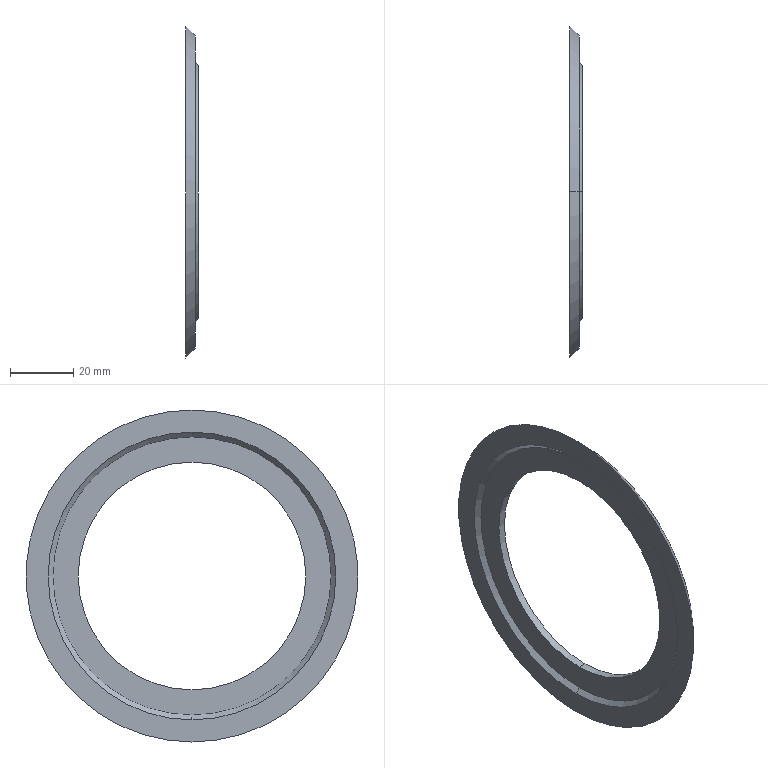Component | SolidWorks | 24Gasket-1 | 1 solid | 12 faces | box 4 x 105 x 105 mm | volume 10058 mm3 | cone 6 | plane 4 | cylinder 2 | commonest cylinder face diameters 72 x2
build123d program:
from build123d import *


with BuildPart() as part:
    # Sketch28 → Revolve1 (revolve)
    with BuildSketch(Plane(origin=(0, 0, 0), x_dir=(0, 0, -1), z_dir=(1, 0, 0)), mode=Mode.PRIVATE) as revolve1_sk:
        Polygon((0, 36), (0, 40), (-1, 41), (-1, 49.5), (-4, 52.5), (-4, 45.5), (-2.5, 44), (-2.5, 36), align=None)
    revolve(revolve1_sk.sketch.rotate(Axis((0, 0, 0), (0, 0, 1)), 90), axis=Axis((0, 0, 0), (0, 0, 1)))


solid = part.part

# Placed as in the assembly
solid = solid.moved(Location((-61.043, 1.776, 250), (0, -90, 0)))
STEP:
#1=CARTESIAN_POINT('',(-2.502,0.06992,11.575));
#2=VERTEX_POINT('',#1);
#3=CARTESIAN_POINT('',(-2.502,0.06992,8.11));
#4=VERTEX_POINT('',#3);
#5=CARTESIAN_POINT('',(-2.502,0.06992,9.843));
#6=DIRECTION('',(1.,0.,0.));
#7=DIRECTION('',(0.,0.,-1.));
#8=AXIS2_PLACEMENT_3D('',#5,#6,#7);
#9=CIRCLE('',#8,1.732);
#10=EDGE_CURVE('',#2,#4,#9,.T.);
#11=ORIENTED_EDGE('',*,*,#10,.T.);
#12=CARTESIAN_POINT('',(-2.561,0.06992,8.051));
#13=VERTEX_POINT('',#12);
#14=CARTESIAN_POINT('',(-2.561,0.06992,8.051));
#15=DIRECTION('',(-0.7071,0.,-0.7071));
#16=VECTOR('',#15,39.37);
#17=LINE('',#14,#16);
#18=EDGE_CURVE('',#4,#13,#17,.T.);
#19=ORIENTED_EDGE('',*,*,#18,.T.);
#20=CARTESIAN_POINT('',(-2.561,0.06992,11.634));
#21=VERTEX_POINT('',#20);
#22=CARTESIAN_POINT('',(-2.561,0.06992,9.843));
#23=DIRECTION('',(1.,0.,0.));
#24=DIRECTION('',(0.,0.,-1.));
#25=AXIS2_PLACEMENT_3D('',#22,#23,#24);
#26=CIRCLE('',#25,1.791);
#27=EDGE_CURVE('',#21,#13,#26,.T.);
#28=ORIENTED_EDGE('',*,*,#27,.F.);
#29=CARTESIAN_POINT('',(-2.561,0.06992,11.634));
#30=DIRECTION('',(-0.7071,0.,0.7071));
#31=VECTOR('',#30,39.37);
#32=LINE('',#29,#31);
#33=EDGE_CURVE('',#2,#21,#32,.T.);
#34=ORIENTED_EDGE('',*,*,#33,.F.);
#35=EDGE_LOOP('',(#11,#19,#28,#34));
#36=FACE_OUTER_BOUND('',#35,.T.);
#37=CARTESIAN_POINT('',(-2.561,0.06992,9.843));
#38=DIRECTION('',(-1.,-0.,-0.));
#39=DIRECTION('',(0.,0.,1.));
#40=AXIS2_PLACEMENT_3D('',#37,#38,#39);
#41=CONICAL_SURFACE('',#40,1.791,0.7854);
#42=ADVANCED_FACE('',(#36),#41,.F.);
#43=CARTESIAN_POINT('',(-2.443,0.06992,7.894));
#44=VERTEX_POINT('',#43);
#45=CARTESIAN_POINT('',(-2.443,0.06992,11.791));
#46=VERTEX_POINT('',#45);
#47=CARTESIAN_POINT('',(-2.443,0.06992,9.843));
#48=DIRECTION('',(1.,0.,0.));
#49=DIRECTION('',(0.,0.,-1.));
#50=AXIS2_PLACEMENT_3D('',#47,#48,#49);
#51=CIRCLE('',#50,1.949);
#52=EDGE_CURVE('',#44,#46,#51,.T.);
#53=ORIENTED_EDGE('',*,*,#52,.F.);
#54=CARTESIAN_POINT('',(-2.561,0.06992,7.776));
#55=VERTEX_POINT('',#54);
#56=CARTESIAN_POINT('',(-2.443,0.06992,7.894));
#57=DIRECTION('',(-0.7071,0.,-0.7071));
#58=VECTOR('',#57,39.37);
#59=LINE('',#56,#58);
#60=EDGE_CURVE('',#44,#55,#59,.T.);
#61=ORIENTED_EDGE('',*,*,#60,.T.);
#62=CARTESIAN_POINT('',(-2.561,0.06992,11.909));
#63=VERTEX_POINT('',#62);
#64=CARTESIAN_POINT('',(-2.561,0.06992,9.843));
#65=DIRECTION('',(1.,0.,0.));
#66=DIRECTION('',(0.,0.,-1.));
#67=AXIS2_PLACEMENT_3D('',#64,#65,#66);
#68=CIRCLE('',#67,2.067);
#69=EDGE_CURVE('',#55,#63,#68,.T.);
#70=ORIENTED_EDGE('',*,*,#69,.T.);
#71=CARTESIAN_POINT('',(-2.443,0.06992,11.791));
#72=DIRECTION('',(-0.7071,0.,0.7071));
#73=VECTOR('',#72,39.37);
#74=LINE('',#71,#73);
#75=EDGE_CURVE('',#46,#63,#74,.T.);
#76=ORIENTED_EDGE('',*,*,#75,.F.);
#77=EDGE_LOOP('',(#53,#61,#70,#76));
#78=FACE_OUTER_BOUND('',#77,.T.);
#79=CARTESIAN_POINT('',(-2.443,0.06992,9.843));
#80=DIRECTION('',(-1.,-0.,-0.));
#81=DIRECTION('',(0.,0.,1.));
#82=AXIS2_PLACEMENT_3D('',#79,#80,#81);
#83=CONICAL_SURFACE('',#82,1.949,0.7854);
#84=ADVANCED_FACE('',(#78),#83,.T.);
#85=CARTESIAN_POINT('',(-2.403,0.06992,8.268));
#86=VERTEX_POINT('',#85);
#87=CARTESIAN_POINT('',(-2.403,0.06992,11.417));
#88=VERTEX_POINT('',#87);
#89=CARTESIAN_POINT('',(-2.403,0.06992,9.843));
#90=DIRECTION('',(1.,0.,0.));
#91=DIRECTION('',(0.,0.,-1.));
#92=AXIS2_PLACEMENT_3D('',#89,#90,#91);
#93=CIRCLE('',#92,1.575);
#94=EDGE_CURVE('',#86,#88,#93,.T.);
#95=ORIENTED_EDGE('',*,*,#94,.F.);
#96=CARTESIAN_POINT('',(-2.443,0.06992,8.228));
#97=VERTEX_POINT('',#96);
#98=CARTESIAN_POINT('',(-2.403,0.06992,8.268));
#99=DIRECTION('',(-0.7071,0.,-0.7071));
#100=VECTOR('',#99,39.37);
#101=LINE('',#98,#100);
#102=EDGE_CURVE('',#86,#97,#101,.T.);
#103=ORIENTED_EDGE('',*,*,#102,.T.);
#104=CARTESIAN_POINT('',(-2.443,0.06992,11.457));
#105=VERTEX_POINT('',#104);
#106=CARTESIAN_POINT('',(-2.443,0.06992,9.843));
#107=DIRECTION('',(1.,0.,0.));
#108=DIRECTION('',(0.,0.,-1.));
#109=AXIS2_PLACEMENT_3D('',#106,#107,#108);
#110=CIRCLE('',#109,1.614);
#111=EDGE_CURVE('',#97,#105,#110,.T.);
#112=ORIENTED_EDGE('',*,*,#111,.T.);
#113=CARTESIAN_POINT('',(-2.403,0.06992,11.417));
#114=DIRECTION('',(-0.7071,0.,0.7071));
#115=VECTOR('',#114,39.37);
#116=LINE('',#113,#115);
#117=EDGE_CURVE('',#88,#105,#116,.T.);
#118=ORIENTED_EDGE('',*,*,#117,.F.);
#119=EDGE_LOOP('',(#95,#103,#112,#118));
#120=FACE_OUTER_BOUND('',#119,.T.);
#121=CARTESIAN_POINT('',(-2.403,0.06992,9.843));
#122=DIRECTION('',(-1.,-0.,-0.));
#123=DIRECTION('',(0.,0.,1.));
#124=AXIS2_PLACEMENT_3D('',#121,#122,#123);
#125=CONICAL_SURFACE('',#124,1.575,0.7854);
#126=ADVANCED_FACE('',(#120),#125,.T.);
#127=CARTESIAN_POINT('',(-2.502,0.06992,11.26));
#128=VERTEX_POINT('',#127);
#129=CARTESIAN_POINT('',(-2.502,0.06992,8.425));
#130=VERTEX_POINT('',#129);
#131=CARTESIAN_POINT('',(-2.502,0.06992,9.843));
#132=DIRECTION('',(1.,0.,0.));
#133=DIRECTION('',(0.,0.,-1.));
#134=AXIS2_PLACEMENT_3D('',#131,#132,#133);
#135=CIRCLE('',#134,1.417);
#136=EDGE_CURVE('',#128,#130,#135,.T.);
#137=ORIENTED_EDGE('',*,*,#136,.F.);
#138=CARTESIAN_POINT('',(-2.403,0.06992,11.26));
#139=VERTEX_POINT('',#138);
#140=CARTESIAN_POINT('',(-2.403,0.06992,11.26));
#141=DIRECTION('',(1.,0.,0.));
#142=VECTOR('',#141,39.37);
#143=LINE('',#140,#142);
#144=EDGE_CURVE('',#128,#139,#143,.T.);
#145=ORIENTED_EDGE('',*,*,#144,.T.);
#146=CARTESIAN_POINT('',(-2.403,0.06992,8.425));
#147=VERTEX_POINT('',#146);
#148=CARTESIAN_POINT('',(-2.403,0.06992,9.843));
#149=DIRECTION('',(1.,0.,0.));
#150=DIRECTION('',(0.,0.,-1.));
#151=AXIS2_PLACEMENT_3D('',#148,#149,#150);
#152=CIRCLE('',#151,1.417);
#153=EDGE_CURVE('',#139,#147,#152,.T.);
#154=ORIENTED_EDGE('',*,*,#153,.T.);
#155=CARTESIAN_POINT('',(-2.403,0.06992,8.425));
#156=DIRECTION('',(1.,0.,0.));
#157=VECTOR('',#156,39.37);
#158=LINE('',#155,#157);
#159=EDGE_CURVE('',#130,#147,#158,.T.);
#160=ORIENTED_EDGE('',*,*,#159,.F.);
#161=EDGE_LOOP('',(#137,#145,#154,#160));
#162=FACE_OUTER_BOUND('',#161,.T.);
#163=CARTESIAN_POINT('',(-2.403,0.06992,9.843));
#164=DIRECTION('',(1.,0.,0.));
#165=DIRECTION('',(0.,0.,-1.));
#166=AXIS2_PLACEMENT_3D('',#163,#164,#165);
#167=CYLINDRICAL_SURFACE('',#166,1.417);
#168=ADVANCED_FACE('',(#162),#167,.F.);
#169=ORIENTED_EDGE('',*,*,#144,.F.);
#170=CARTESIAN_POINT('',(-2.502,0.06992,9.843));
#171=DIRECTION('',(1.,0.,0.));
#172=DIRECTION('',(0.,0.,-1.));
#173=AXIS2_PLACEMENT_3D('',#170,#171,#172);
#174=CIRCLE('',#173,1.417);
#175=EDGE_CURVE('',#130,#128,#174,.T.);
#176=ORIENTED_EDGE('',*,*,#175,.F.);
#177=ORIENTED_EDGE('',*,*,#159,.T.);
#178=CARTESIAN_POINT('',(-2.403,0.06992,9.843));
#179=DIRECTION('',(1.,0.,0.));
#180=DIRECTION('',(0.,0.,-1.));
#181=AXIS2_PLACEMENT_3D('',#178,#179,#180);
#182=CIRCLE('',#181,1.417);
#183=EDGE_CURVE('',#147,#139,#182,.T.);
#184=ORIENTED_EDGE('',*,*,#183,.T.);
#185=EDGE_LOOP('',(#169,#176,#177,#184));
#186=FACE_OUTER_BOUND('',#185,.T.);
#187=CARTESIAN_POINT('',(-2.403,0.06992,9.843));
#188=DIRECTION('',(1.,0.,0.));
#189=DIRECTION('',(0.,0.,-1.));
#190=AXIS2_PLACEMENT_3D('',#187,#188,#189);
#191=CYLINDRICAL_SURFACE('',#190,1.417);
#192=ADVANCED_FACE('',(#186),#191,.F.);
#193=CARTESIAN_POINT('',(-2.403,0.06992,9.843));
#194=DIRECTION('',(1.,0.,0.));
#195=DIRECTION('',(0.,0.,-1.));
#196=AXIS2_PLACEMENT_3D('',#193,#194,#195);
#197=CIRCLE('',#196,1.575);
#198=EDGE_CURVE('',#88,#86,#197,.T.);
#199=ORIENTED_EDGE('',*,*,#198,.T.);
#200=ORIENTED_EDGE('',*,*,#94,.T.);
#201=EDGE_LOOP('',(#199,#200));
#202=FACE_OUTER_BOUND('',#201,.T.);
#203=ORIENTED_EDGE('',*,*,#183,.F.);
#204=ORIENTED_EDGE('',*,*,#153,.F.);
#205=EDGE_LOOP('',(#203,#204));
#206=FACE_BOUND('',#205,.T.);
#207=CARTESIAN_POINT('',(-2.403,1.487,9.843));
#208=DIRECTION('',(1.,0.,0.));
#209=DIRECTION('',(0.,-0.,-1.));
#210=AXIS2_PLACEMENT_3D('',#207,#208,#209);
#211=PLANE('',#210);
#212=ADVANCED_FACE('',(#202,#206),#211,.T.);
#213=ORIENTED_EDGE('',*,*,#102,.F.);
#214=ORIENTED_EDGE('',*,*,#198,.F.);
#215=ORIENTED_EDGE('',*,*,#117,.T.);
#216=CARTESIAN_POINT('',(-2.443,0.06992,9.843));
#217=DIRECTION('',(1.,0.,0.));
#218=DIRECTION('',(0.,0.,-1.));
#219=AXIS2_PLACEMENT_3D('',#216,#217,#218);
#220=CIRCLE('',#219,1.614);
#221=EDGE_CURVE('',#105,#97,#220,.T.);
#222=ORIENTED_EDGE('',*,*,#221,.T.);
#223=EDGE_LOOP('',(#213,#214,#215,#222));
#224=FACE_OUTER_BOUND('',#223,.T.);
#225=CARTESIAN_POINT('',(-2.403,0.06992,9.843));
#226=DIRECTION('',(-1.,-0.,-0.));
#227=DIRECTION('',(0.,0.,1.));
#228=AXIS2_PLACEMENT_3D('',#225,#226,#227);
#229=CONICAL_SURFACE('',#228,1.575,0.7854);
#230=ADVANCED_FACE('',(#224),#229,.T.);
#231=CARTESIAN_POINT('',(-2.443,0.06992,9.843));
#232=DIRECTION('',(1.,0.,0.));
#233=DIRECTION('',(0.,0.,-1.));
#234=AXIS2_PLACEMENT_3D('',#231,#232,#233);
#235=CIRCLE('',#234,1.949);
#236=EDGE_CURVE('',#46,#44,#235,.T.);
#237=ORIENTED_EDGE('',*,*,#236,.T.);
#238=ORIENTED_EDGE('',*,*,#52,.T.);
#239=EDGE_LOOP('',(#237,#238));
#240=FACE_OUTER_BOUND('',#239,.T.);
#241=ORIENTED_EDGE('',*,*,#221,.F.);
#242=ORIENTED_EDGE('',*,*,#111,.F.);
#243=EDGE_LOOP('',(#241,#242));
#244=FACE_BOUND('',#243,.T.);
#245=CARTESIAN_POINT('',(-2.443,1.684,9.843));
#246=DIRECTION('',(1.,0.,0.));
#247=DIRECTION('',(0.,-0.,-1.));
#248=AXIS2_PLACEMENT_3D('',#245,#246,#247);
#249=PLANE('',#248);
#250=ADVANCED_FACE('',(#240,#244),#249,.T.);
#251=ORIENTED_EDGE('',*,*,#60,.F.);
#252=ORIENTED_EDGE('',*,*,#236,.F.);
#253=ORIENTED_EDGE('',*,*,#75,.T.);
#254=CARTESIAN_POINT('',(-2.561,0.06992,9.843));
#255=DIRECTION('',(1.,0.,0.));
#256=DIRECTION('',(0.,0.,-1.));
#257=AXIS2_PLACEMENT_3D('',#254,#255,#256);
#258=CIRCLE('',#257,2.067);
#259=EDGE_CURVE('',#63,#55,#258,.T.);
#260=ORIENTED_EDGE('',*,*,#259,.T.);
#261=EDGE_LOOP('',(#251,#252,#253,#260));
#262=FACE_OUTER_BOUND('',#261,.T.);
#263=CARTESIAN_POINT('',(-2.443,0.06992,9.843));
#264=DIRECTION('',(-1.,-0.,-0.));
#265=DIRECTION('',(0.,0.,1.));
#266=AXIS2_PLACEMENT_3D('',#263,#264,#265);
#267=CONICAL_SURFACE('',#266,1.949,0.7854);
#268=ADVANCED_FACE('',(#262),#267,.T.);
#269=ORIENTED_EDGE('',*,*,#27,.T.);
#270=CARTESIAN_POINT('',(-2.561,0.06992,9.843));
#271=DIRECTION('',(1.,0.,0.));
#272=DIRECTION('',(0.,0.,-1.));
#273=AXIS2_PLACEMENT_3D('',#270,#271,#272);
#274=CIRCLE('',#273,1.791);
#275=EDGE_CURVE('',#13,#21,#274,.T.);
#276=ORIENTED_EDGE('',*,*,#275,.T.);
#277=EDGE_LOOP('',(#269,#276));
#278=FACE_BOUND('',#277,.T.);
#279=ORIENTED_EDGE('',*,*,#259,.F.);
#280=ORIENTED_EDGE('',*,*,#69,.F.);
#281=EDGE_LOOP('',(#279,#280));
#282=FACE_OUTER_BOUND('',#281,.T.);
#283=CARTESIAN_POINT('',(-2.561,2.137,9.843));
#284=DIRECTION('',(-1.,-0.,-0.));
#285=DIRECTION('',(-0.,0.,1.));
#286=AXIS2_PLACEMENT_3D('',#283,#284,#285);
#287=PLANE('',#286);
#288=ADVANCED_FACE('',(#278,#282),#287,.T.);
#289=ORIENTED_EDGE('',*,*,#18,.F.);
#290=CARTESIAN_POINT('',(-2.502,0.06992,9.843));
#291=DIRECTION('',(1.,0.,0.));
#292=DIRECTION('',(0.,0.,-1.));
#293=AXIS2_PLACEMENT_3D('',#290,#291,#292);
#294=CIRCLE('',#293,1.732);
#295=EDGE_CURVE('',#4,#2,#294,.T.);
#296=ORIENTED_EDGE('',*,*,#295,.T.);
#297=ORIENTED_EDGE('',*,*,#33,.T.);
#298=ORIENTED_EDGE('',*,*,#275,.F.);
#299=EDGE_LOOP('',(#289,#296,#297,#298));
#300=FACE_OUTER_BOUND('',#299,.T.);
#301=CARTESIAN_POINT('',(-2.561,0.06992,9.843));
#302=DIRECTION('',(-1.,-0.,-0.));
#303=DIRECTION('',(0.,0.,1.));
#304=AXIS2_PLACEMENT_3D('',#301,#302,#303);
#305=CONICAL_SURFACE('',#304,1.791,0.7854);
#306=ADVANCED_FACE('',(#300),#305,.F.);
#307=ORIENTED_EDGE('',*,*,#175,.T.);
#308=ORIENTED_EDGE('',*,*,#136,.T.);
#309=EDGE_LOOP('',(#307,#308));
#310=FACE_BOUND('',#309,.T.);
#311=ORIENTED_EDGE('',*,*,#10,.F.);
#312=ORIENTED_EDGE('',*,*,#295,.F.);
#313=EDGE_LOOP('',(#311,#312));
#314=FACE_OUTER_BOUND('',#313,.T.);
#315=CARTESIAN_POINT('',(-2.502,1.802,9.843));
#316=DIRECTION('',(-1.,-0.,-0.));
#317=DIRECTION('',(-0.,0.,1.));
#318=AXIS2_PLACEMENT_3D('',#315,#316,#317);
#319=PLANE('',#318);
#320=ADVANCED_FACE('',(#310,#314),#319,.T.);
#321=CLOSED_SHELL('',(#42,#84,#126,#168,#192,#212,#230,#250,#268,#288,#306,#320));
#322=MANIFOLD_SOLID_BREP('',#321);
#323=CARTESIAN_POINT('',(0.,0.,0.));
#324=DIRECTION('',(0.,0.,1.));
#325=DIRECTION('',(1.,0.,0.));
#326=AXIS2_PLACEMENT_3D('',#323,#324,#325);
#327=(LENGTH_UNIT()NAMED_UNIT(*)SI_UNIT($,.METRE.));
#328=LENGTH_MEASURE_WITH_UNIT(LENGTH_MEASURE(0.0254),#327);
#329=DIMENSIONAL_EXPONENTS(1.,0.,0.,0.,0.,0.,0.);
#330=(CONVERSION_BASED_UNIT('',#328)LENGTH_UNIT()NAMED_UNIT(#329));
#331=UNCERTAINTY_MEASURE_WITH_UNIT(LENGTH_MEASURE(0.00001),#330,'','');
#332=(NAMED_UNIT(*)PLANE_ANGLE_UNIT()SI_UNIT($,.RADIAN.));
#333=(NAMED_UNIT(*)SI_UNIT($,.STERADIAN.)SOLID_ANGLE_UNIT());
#334=(GEOMETRIC_REPRESENTATION_CONTEXT(3)GLOBAL_UNCERTAINTY_ASSIGNED_CONTEXT((#331))GLOBAL_UNIT_ASSIGNED_CONTEXT((#330,#332,#333))REPRESENTATION_CONTEXT('',''));
#335=ADVANCED_BREP_SHAPE_REPRESENTATION('',(#322,#326),#334);
#336=COLOUR_RGB('',0.7922,0.8196,0.9333);
#337=FILL_AREA_STYLE_COLOUR('',#336);
#338=FILL_AREA_STYLE('',(#337));
#339=SURFACE_STYLE_FILL_AREA(#338);
#340=SURFACE_SIDE_STYLE('',(#339));
#341=SURFACE_STYLE_USAGE(.BOTH.,#340);
#342=PRESENTATION_STYLE_ASSIGNMENT((#341));
#343=STYLED_ITEM('',(#342),#322);
#344=(LENGTH_UNIT()NAMED_UNIT(*)SI_UNIT($,.METRE.));
#345=LENGTH_MEASURE_WITH_UNIT(LENGTH_MEASURE(0.0254),#344);
#346=DIMENSIONAL_EXPONENTS(1.,0.,0.,0.,0.,0.,0.);
#347=(CONVERSION_BASED_UNIT('',#345)LENGTH_UNIT()NAMED_UNIT(#346));
#348=UNCERTAINTY_MEASURE_WITH_UNIT(LENGTH_MEASURE(0.00001),#347,'','');
#349=(NAMED_UNIT(*)PLANE_ANGLE_UNIT()SI_UNIT($,.RADIAN.));
#350=(NAMED_UNIT(*)SI_UNIT($,.STERADIAN.)SOLID_ANGLE_UNIT());
#351=(GEOMETRIC_REPRESENTATION_CONTEXT(3)GLOBAL_UNCERTAINTY_ASSIGNED_CONTEXT((#348))GLOBAL_UNIT_ASSIGNED_CONTEXT((#347,#349,#350))REPRESENTATION_CONTEXT('',''));
#352=MECHANICAL_DESIGN_GEOMETRIC_PRESENTATION_REPRESENTATION('',(#343),#351);
#353=PRESENTATION_LAYER_ASSIGNMENT('','',(#343));